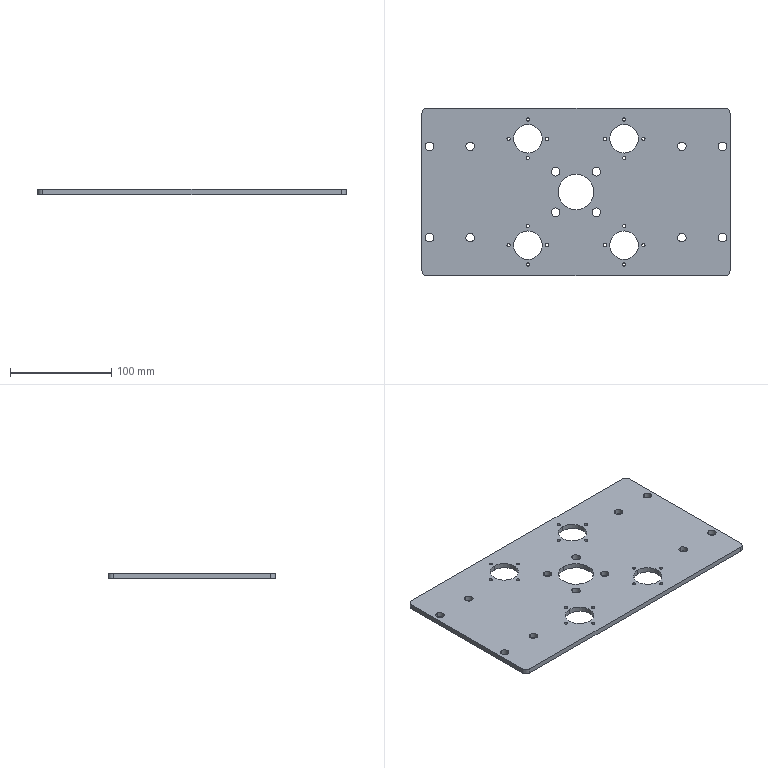Component | SolidWorks | DC-46-014-4 | 1 solid | 76 faces | box 304 x 165 x 5 mm | volume 229302 mm3 | cylinder 70 | plane 6 | commonest cylinder face diameters 3.3 x32 8.5 x24 28.2 x8 10 x4 35 x2
build123d program:
from build123d import *

# Parameters (mm, degrees)
SKETCH1_W                  = 165
SKETCH1_H                  = 304
BOSS_EXTRUDE1_DEPTH        = 2.5
FILLET1_R                  = 5
F_8_5_8_5_DIAMETER_HOLE1_D = 8.5
SKETCH4_R                  = 17.5
CUT_EXTRUDE1_DEPTH         = 82
F_8_5_8_5_DIAMETER_HOLE2_D = 8.5
SKETCH7_R                  = 14.1
CUT_EXTRUDE2_DEPTH         = 82
M4_TAPPED_HOLE1_D          = 3.3


with BuildPart() as part:
    # Sketch1 → Boss-Extrude1 (new, symmetric)
    with BuildSketch(Plane.XY):
        Rectangle(SKETCH1_W, SKETCH1_H)
    extrude(amount=BOSS_EXTRUDE1_DEPTH, both=True)

    # Fillet1
    fillet1_edges = [part.edges().sort_by_distance(p)[0] for p in [
        (-82.5, 152, 0),
        (82.5, 152, 0),
        (82.5, -152, 0),
        (-82.5, -152, 0),
    ]]
    fillet(fillet1_edges, radius=FILLET1_R)

    # 8.5 _8.5_ Diameter Hole1 (through all)
    with Locations(Plane.XY.offset(2.5)):
        with Locations((-45, 144.5), (45, 144.5), (45, 104.5), (-45, 104.5), (45, -144.5), (45, -104.5), (-45, -104.5), (-45, -144.5)):
            Hole(F_8_5_8_5_DIAMETER_HOLE1_D / 2)

    # Sketch4 → Cut-Extrude1 (cut)
    with BuildSketch(Plane.XY.offset(2.5)):
        Circle(SKETCH4_R)
    extrude(amount=-CUT_EXTRUDE1_DEPTH, mode=Mode.SUBTRACT)

    # 8.5 _8.5_ Diameter Hole2 (through all)
    with Locations(Plane(origin=(0, 0, -2.5), x_dir=(-1, 0, 0), z_dir=(0, 0, -1))):
        with Locations((20, -20), (20, 20), (-20, 20), (-20, -20)):
            Hole(F_8_5_8_5_DIAMETER_HOLE2_D / 2)

    # Sketch7 → Cut-Extrude2 (cut)
    with BuildSketch(Plane(origin=(0, 0, -2.5), x_dir=(-1, 0, 0), z_dir=(0, 0, -1))):
        with Locations((52.5, -47.5)):
            Circle(SKETCH7_R)
        with Locations((-52.5, -47.5)):
            Circle(SKETCH7_R)
        with Locations((52.5, 47.5)):
            Circle(SKETCH7_R)
        with Locations((-52.5, 47.5)):
            Circle(SKETCH7_R)
    extrude(amount=-CUT_EXTRUDE2_DEPTH, mode=Mode.SUBTRACT)

    # M4 Tapped Hole1 (through all)
    with Locations(Plane.XY.offset(2.5)):
        with Locations((52.5, -66.5), (71.5, -47.5), (33.5, -47.5), (52.5, -28.5), (52.5, 66.5), (33.5, 47.5), (52.5, 28.5), (71.5, 47.5), (-52.5, 28.5), (-33.5, 47.5), (-52.5, 66.5), (-71.5, 47.5), (-52.5, -66.5), (-33.5, -47.5), (-52.5, -28.5), (-71.5, -47.5)):
            Hole(M4_TAPPED_HOLE1_D / 2)


solid = part.part

# Placed as in the assembly
solid = solid.moved(Location((311.865, 195.227, 2029.633), (0, 0, 90)))